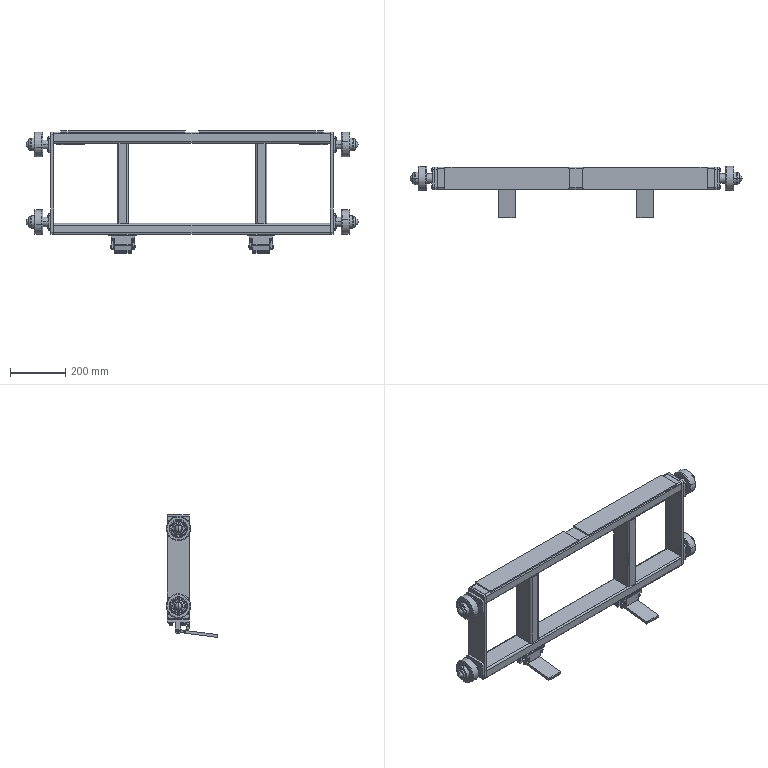Assembly | SolidWorks | mm | 114 component files | 114 solids | 2486 faces | box 1200 x 186.22 x 443.19 mm | volume 4209705 mm3 | cylinder 894 | plane 856 | torus 336 | sphere 224 | cone 176 | commonest cylinder face diameters 10 x84 8 x80 6 x80 4 x52 6.5 x48 9.684 x48 16 x40 11 x32
Bill of materials:
GB_T70.1-2000_SocketHeadCapScrew_M6_16 | 16 |  | Headed pin or screw-like body: a short, larger-diameter cylindrical head joined to a longer, smaller-diameter plain cylindrical shank that has a chamfered free end.
GB_T70.1-2000_SocketHeadCapScrew_M8_25 | 8 |  | Headed cylindrical body: a short, wide cylindrical head with a longer, narrower plain cylindrical shank that has a chamfered end. The shape is very close to the previous part, with slightly different proportions.
GB_T93-1987StandardTypeSpringWasher(Assembly)6x1.6 | 16 |  | Split ring with a rectangular cross-section and a single radial gap. Its radial width is fairly large compared with its thickness, which suggests a split-washer shape.
GB_T93-1987StandardTypeSpringWasher(Assembly)8x2.1 | 8 |  | Flat split ring: a thin annulus with one narrow radial slot cut through it, and a rectangular cross-section.
GB_T97.2-1985FlatWasherChamferedTypeA8x1.6 | 8 | Steel | Flat washer-like annulus: a thin disc with a central circular hole, chamfered on one outer edge.
GB_T276-94DeepGrooveBallBearing6305-2Z | 4 |  | Ring assembly-like solid that looks like a radial ball bearing: concentric outer and inner rings with a central bore, and several spherical elements visible in the annular gap between them.
GB893.2-86RetainingRingForHolesTypeB62 | 4 |  | Thin open ring shaped like an internal retaining ring: a circular band with an opening at one side, ending in two widened lugs that each have a small hole.
GuideWheel | 4 | Nylon 101 | Plain thick ring or sleeve: a wide annulus with a large central bore and rounded outer edges.
GuideWheelAxis | 4 | Q235 | Stepped solid cylinder or shaft: a larger-diameter central section with smaller-diameter end sections on both sides, one longer than the other, both with chamfered ends.
GuideWheelBracketPlate | 4 | Q235 | Flat rectangular plate with rounded corners, a large central circular through hole, and four smaller through holes near the corners.
WD-03UniversalBall | 4 |  | Compound axisymmetric body: a domed or hemispherical end, a stepped cylindrical housing with a wider collar band, and a small cylindrical pin with a chamfered tip projecting from the opposite face.
AWS5_30 | 4 |  | Long, thin-walled hollow cylindrical body with an open, nearly circular round-wire hook loop at each end. The hooks sit on the body axis and look like they lie in the same plane. Overall it looks like a simplified extension spring with the coils drawn as a smooth tube.
GB_T70.1-2000_SocketHeadCapScrew_M4_12 | 8 |  | Socket-head-style headed body: a cylindrical head with a hexagonal recess in its end face, and a plain cylindrical shank with a chamfered tip.
GB_T78-2000HexagonSocketConePointSetScrewM4x6 | 4 |  | Short solid cylinder with a conical top that ends in a small flat circular tip and a chamfer around the bottom edge.
LiftingPlate | 2 | Plain Carbon Steel | Flat rectangular leaf with a hollow cylindrical knuckle (bored boss) along one edge and a small hole near the knuckle. The free end is slightly rounded.
LiftingPlateAxis | 2 | Plain Carbon Steel | Straight solid cylindrical rod or pin with small chamfers at both ends.
LiftingPlateBracket | 2 | Plain Carbon Steel | Bracket block: a rectangular top plate with four corner through holes and downward legs or lugs below it. One lug has a large cross bore and chamfered lower corners. A narrower leg has a small conical-bottom hole.
RectangularTubeEndPlate | 2 | Plain Carbon Steel | Thin, elongated rectangular plate with rounded corners and eight small holes arranged in two groups of four, one group near each end.
RectangularTubeWeldPlate1 | 2 | Plain Carbon Steel | Flat rectangular plate, close to square, with rounded corners and four through holes near the corners.
RectangularTubeWeldPlate2 | 2 | Plain Carbon Steel | Thin, long rectangular strip or plate with small rounded corners and no holes.
RectangularTubeWeldPlate3 | 2 | Plain Carbon Steel | Flat rectangular plate with rounded corners and four through holes near the corners. It is more elongated than unnamed part.
VerticalMovingRectangularTube | 2 | Plain Carbon Steel | Long, straight, hollow rectangular tube with rounded corners and a thin uniform wall. The ends are cut square.
VerticalMovingTube | 2 | Plain Carbon Steel | Short, hollow rectangular tube with rounded corners and a thin uniform wall. The cross-section is about 1:2 and the ends are open and cut square.
Mates:
1. coincident | VerticalMovingRectangularTubeWeldment-1/RectangularTubeWeldPlate1-1 face at (510, 56.339, -25) dir (0, 0, -1) | LiftingPlateAssembly-1/LiftingPlateBracket-1 face at (-207.5, -40, -25) dir (0, 0, 1)
2. concentric | VerticalMovingRectangularTubeWeldment-1/RectangularTubeWeldPlate1-1 face at (-280, 27.5, -25) dir (0, 0, -1) r 4 | LiftingPlateAssembly-1/LiftingPlateBracket-1 face at (-280, 27.5, -35) dir (0, 0, -1) r 4.5
3. concentric | VerticalMovingRectangularTubeWeldment-1/RectangularTubeWeldPlate1-1 face at (-220, -19, -25) dir (0, 0, -1) r 4 | LiftingPlateAssembly-1/LiftingPlateBracket-1 face at (-220, -19, -35) dir (0, 0, -1) r 4.5
4. coincident | VerticalMovingRectangularTubeWeldment-1/RectangularTubeWeldPlate1-2 face at (510, 56.339, -25) dir (0, 0, -1) | LiftingPlateAssembly-2/LiftingPlateBracket-1 face at (292.5, -40, -25) dir (0, 0, 1)
5. concentric | VerticalMovingRectangularTubeWeldment-1/RectangularTubeWeldPlate1-2 face at (220, 27.5, -25) dir (0, 0, -1) r 4 | LiftingPlateAssembly-2/LiftingPlateBracket-1 face at (220, 27.5, -35) dir (0, 0, -1) r 4.5
6. concentric | VerticalMovingRectangularTubeWeldment-1/RectangularTubeWeldPlate1-2 face at (280, -19, -25) dir (0, 0, -1) r 4 | LiftingPlateAssembly-2/LiftingPlateBracket-1 face at (280, -19, -35) dir (0, 0, -1) r 4.5
7. coincident | VerticalMovingRectangularTubeWeldment-1/RectangularTubeEndPlate-1 face at (-510, 0, 165) dir (-1, 0, 0) | GuideWheelAssembly-1/GuideWheelBracket-1/GuideWheelBracketPlate-1 face at (-510, 0, 25) dir (1, 0, 0)
8. concentric | VerticalMovingRectangularTubeWeldment-1/RectangularTubeEndPlate-1 face at (-510, 30, 5) dir (-1, 0, 0) r 3 | GuideWheelAssembly-1/GuideWheelBracket-1/GuideWheelBracketPlate-1 face at (-520, 30, 5) dir (-1, 0, 0) r 5.5
9. concentric | VerticalMovingRectangularTubeWeldment-1/RectangularTubeEndPlate-1 face at (-510, -30, 45) dir (-1, 0, 0) r 3 | GuideWheelAssembly-1/GuideWheelBracket-1/GuideWheelBracketPlate-1 face at (-520, -30, 45) dir (-1, 0, 0) r 5.5
10. coincident | VerticalMovingRectangularTubeWeldment-1/RectangularTubeEndPlate-1 face at (-510, 0, 165) dir (-1, 0, 0) | GuideWheelAssembly-2/GuideWheelBracket-1/GuideWheelBracketPlate-1 face at (-510, 0, 305) dir (1, 0, 0)
11. concentric | VerticalMovingRectangularTubeWeldment-1/RectangularTubeEndPlate-1 face at (-510, 30, 325) dir (-1, 0, 0) r 3 | GuideWheelAssembly-2/GuideWheelBracket-1/GuideWheelBracketPlate-1 face at (-520, 30, 325) dir (-1, 0, 0) r 5.5
12. concentric | VerticalMovingRectangularTubeWeldment-1/RectangularTubeEndPlate-1 face at (-510, -30, 285) dir (-1, 0, 0) r 3 | GuideWheelAssembly-2/GuideWheelBracket-1/GuideWheelBracketPlate-1 face at (-520, -30, 285) dir (-1, 0, 0) r 5.5
13. coincident | VerticalMovingRectangularTubeWeldment-1/RectangularTubeEndPlate-2 face at (510, 0, 165) dir (1, 0, 0) | GuideWheelAssembly-3/GuideWheelBracket-1/GuideWheelBracketPlate-1 face at (510, 0, 25) dir (-1, 0, 0)
14. concentric | VerticalMovingRectangularTubeWeldment-1/RectangularTubeEndPlate-2 face at (510, 30, 45) dir (1, 0, 0) r 3 | GuideWheelAssembly-3/GuideWheelBracket-1/GuideWheelBracketPlate-1 face at (520, 30, 45) dir (1, 0, 0) r 5.5
15. concentric | VerticalMovingRectangularTubeWeldment-1/RectangularTubeEndPlate-2 face at (510, -30, 5) dir (1, 0, 0) r 3 | GuideWheelAssembly-3/GuideWheelBracket-1/GuideWheelBracketPlate-1 face at (520, -30, 5) dir (1, 0, 0) r 5.5
16. coincident | VerticalMovingRectangularTubeWeldment-1/RectangularTubeEndPlate-2 face at (510, 0, 165) dir (1, 0, 0) | GuideWheelAssembly-4/GuideWheelBracket-1/GuideWheelBracketPlate-1 face at (510, 0, 305) dir (-1, 0, 0)
17. concentric | VerticalMovingRectangularTubeWeldment-1/RectangularTubeEndPlate-2 face at (510, 30, 325) dir (1, 0, 0) r 3 | GuideWheelAssembly-4/GuideWheelBracket-1/GuideWheelBracketPlate-1 face at (520, 30, 325) dir (1, 0, 0) r 5.5
18. concentric | VerticalMovingRectangularTubeWeldment-1/RectangularTubeEndPlate-2 face at (510, -30, 285) dir (1, 0, 0) r 3 | GuideWheelAssembly-4/GuideWheelBracket-1/GuideWheelBracketPlate-1 face at (520, -30, 285) dir (1, 0, 0) r 5.5
19. coincident | GuideWheelAssembly-2/GuideWheelBracket-1/GuideWheelBracketPlate-1 face at (-513.2, 26.7, 325) dir (-1, 0, 0) | GB_T93-1987StandardTypeSpringWasher(Assembly)6x1.6-1 face at (-513.2, 30, 325) dir (1, 0, 0)
20. coincident | GuideWheelAssembly-2/GuideWheelBracket-1/GuideWheelBracketPlate-1 face at (-513.2, 26.7, 325) dir (-1, 0, 0) | GB_T93-1987StandardTypeSpringWasher(Assembly)6x1.6-15 face at (-513.2, -30, 325) dir (1, 0, 0)
21. concentric | GuideWheelAssembly-2/GuideWheelBracket-1/GuideWheelBracketPlate-1 face at (-520, 30, 325) dir (-1, 0, 0) r 5.5 | GB_T93-1987StandardTypeSpringWasher(Assembly)6x1.6-1 face at (-513.2, 30, 325) dir (-1, 0, 0) r 3.25
22. concentric | GuideWheelAssembly-2/GuideWheelBracket-1/GuideWheelBracketPlate-1 face at (-520, -30, 325) dir (-1, 0, 0) r 5.5 | GB_T93-1987StandardTypeSpringWasher(Assembly)6x1.6-15 face at (-513.2, -30, 325) dir (-1, 0, 0) r 3.25
23. coincident | GuideWheelAssembly-4/GuideWheelBracket-1/GuideWheelBracketPlate-1 face at (513.2, 33.3, 325) dir (1, 0, 0) | GB_T93-1987StandardTypeSpringWasher(Assembly)6x1.6-19 face at (513.2, 30, 325) dir (-1, 0, 0)
24. coincident | GuideWheelAssembly-4/GuideWheelBracket-1/GuideWheelBracketPlate-1 face at (513.2, 33.3, 325) dir (1, 0, 0) | GB_T93-1987StandardTypeSpringWasher(Assembly)6x1.6-23 face at (513.2, -30, 325) dir (-1, 0, 0)
25. concentric | GuideWheelAssembly-4/GuideWheelBracket-1/GuideWheelBracketPlate-1 face at (520, 30, 325) dir (1, 0, 0) r 5.5 | GB_T93-1987StandardTypeSpringWasher(Assembly)6x1.6-19 face at (513.2, 30, 325) dir (1, 0, 0) r 3.25
26. concentric | GuideWheelAssembly-4/GuideWheelBracket-1/GuideWheelBracketPlate-1 face at (520, -30, 325) dir (1, 0, 0) r 5.5 | GB_T93-1987StandardTypeSpringWasher(Assembly)6x1.6-23 face at (513.2, -30, 325) dir (1, 0, 0) r 3.25
27. coincident | GB_T93-1987StandardTypeSpringWasher(Assembly)6x1.6-1 face at (-514.8, 30, 325) dir (-1, 0, 0) | GB_T70.1-2000_SocketHeadCapScrew_M6_16-15 face at (-514.8, 35, 325) dir (1, 0, 0)
28. coincident | GB_T70.1-2000_SocketHeadCapScrew_M6_16-1 face at (-514.8, -25, 325) dir (1, 0, 0) | GB_T70.1-2000_SocketHeadCapScrew_M6_16-15 face at (-514.8, 35, 325) dir (1, 0, 0)
29. concentric | GuideWheelAssembly-2/GuideWheelBracket-1/GuideWheelBracketPlate-1 face at (-520, 30, 325) dir (-1, 0, 0) r 5.5 | GB_T70.1-2000_SocketHeadCapScrew_M6_16-15 face at (-520.8, 30, 325) dir (-1, 0, 0) r 3
30. concentric | GuideWheelAssembly-2/GuideWheelBracket-1/GuideWheelBracketPlate-1 face at (-520, -30, 325) dir (-1, 0, 0) r 5.5 | GB_T70.1-2000_SocketHeadCapScrew_M6_16-1 face at (-520.8, -30, 325) dir (-1, 0, 0) r 3
31. coincident | GB_T93-1987StandardTypeSpringWasher(Assembly)6x1.6-23 face at (514.8, -30, 325) dir (1, 0, 0) | GB_T70.1-2000_SocketHeadCapScrew_M6_16-19 face at (514.8, 31.909, 320.379) dir (-1, 0, 0)
32. coincident | GB_T93-1987StandardTypeSpringWasher(Assembly)6x1.6-23 face at (514.8, -30, 325) dir (1, 0, 0) | GB_T70.1-2000_SocketHeadCapScrew_M6_16-23 face at (514.8, -28.091, 320.379) dir (-1, 0, 0)
33. concentric | GuideWheelAssembly-4/GuideWheelBracket-1/GuideWheelBracketPlate-1 face at (520, -30, 325) dir (1, 0, 0) r 5.5 | GB_T70.1-2000_SocketHeadCapScrew_M6_16-23 face at (520.8, -30, 325) dir (1, 0, 0) r 3
34. concentric | GuideWheelAssembly-4/GuideWheelBracket-1/GuideWheelBracketPlate-1 face at (520, 30, 325) dir (1, 0, 0) r 5.5 | GB_T70.1-2000_SocketHeadCapScrew_M6_16-19 face at (520.8, 30, 325) dir (1, 0, 0) r 3
35. coincident | LiftingPlateAssembly-1/LiftingPlateBracket-1 face at (-207.5, 12, -35) dir (0, 0, -1) | GB_T97.2-1985FlatWasherChamferedTypeA8x1.6-13 face at (-284.2, -19, -35) dir (0, 0, 1)
36. coincident | LiftingPlateAssembly-1/LiftingPlateBracket-1 face at (-207.5, -8, -35) dir (0, 0, -1) | GB_T97.2-1985FlatWasherChamferedTypeA8x1.6-11 face at (-224.2, 27.5, -35) dir (0, 0, 1)
37. coincident | LiftingPlateAssembly-1/LiftingPlateBracket-1 face at (-207.5, -8, -35) dir (0, 0, -1) | GB_T97.2-1985FlatWasherChamferedTypeA8x1.6-9 face at (-224.2, -19, -35) dir (0, 0, 1)
38. coincident | LiftingPlateAssembly-1/LiftingPlateBracket-1 face at (-207.5, -8, -35) dir (0, 0, -1) | GB_T97.2-1985FlatWasherChamferedTypeA8x1.6-1 face at (-284.2, 27.5, -35) dir (0, 0, 1)
39. concentric | LiftingPlateAssembly-1/LiftingPlateBracket-1 face at (-280, -19, -35) dir (0, 0, -1) r 4.5 | GB_T97.2-1985FlatWasherChamferedTypeA8x1.6-13 face at (-280, -19, -26.355) dir (0, 0, 1) r 4.2
40. concentric | LiftingPlateAssembly-1/LiftingPlateBracket-1 face at (-280, 27.5, -35) dir (0, 0, -1) r 4.5 | GB_T97.2-1985FlatWasherChamferedTypeA8x1.6-1 face at (-280, 27.5, -26.355) dir (0, 0, 1) r 4.2
41. concentric | LiftingPlateAssembly-1/LiftingPlateBracket-1 face at (-220, 27.5, -35) dir (0, 0, -1) r 4.5 | GB_T97.2-1985FlatWasherChamferedTypeA8x1.6-11 face at (-220, 27.5, -26.355) dir (0, 0, 1) r 4.2
42. concentric | LiftingPlateAssembly-1/LiftingPlateBracket-1 edge at (-220, -19, -35) dir (0, 0, -1) r 4.5 | GB_T97.2-1985FlatWasherChamferedTypeA8x1.6-9 face at (-220, -19, -26.355) dir (0, 0, 1) r 4.2
43. coincident | GB_T97.2-1985FlatWasherChamferedTypeA8x1.6-13 face at (-284.2, -19, -36.6) dir (0, 0, -1) | GB_T93-1987StandardTypeSpringWasher(Assembly)8x2.1-8 face at (-280, -19, -36.6) dir (0, 0, 1)
44. coincident | GB_T93-1987StandardTypeSpringWasher(Assembly)8x2.1-6 face at (-220, 27.5, -36.6) dir (0, 0, 1) | GB_T93-1987StandardTypeSpringWasher(Assembly)8x2.1-8 face at (-280, -19, -36.6) dir (0, 0, 1)
45. coincident | GB_T93-1987StandardTypeSpringWasher(Assembly)8x2.1-8 face at (-280, -19, -36.6) dir (0, 0, 1) | GB_T93-1987StandardTypeSpringWasher(Assembly)8x2.1-10 face at (-280, 27.5, -36.6) dir (0, 0, 1)
46. coincident | GB_T93-1987StandardTypeSpringWasher(Assembly)8x2.1-1 face at (-220, -19, -36.6) dir (0, 0, 1) | GB_T93-1987StandardTypeSpringWasher(Assembly)8x2.1-6 face at (-220, 27.5, -36.6) dir (0, 0, 1)
47. concentric | GB_T97.2-1985FlatWasherChamferedTypeA8x1.6-11 face at (-220, 27.5, -26.355) dir (0, 0, 1) r 4.2 | GB_T93-1987StandardTypeSpringWasher(Assembly)8x2.1-6 face at (-220, 27.5, -36.6) dir (0, 0, -1) r 4.25
48. concentric | GB_T97.2-1985FlatWasherChamferedTypeA8x1.6-1 face at (-280, 27.5, -26.355) dir (0, 0, 1) r 4.2 | GB_T93-1987StandardTypeSpringWasher(Assembly)8x2.1-10 face at (-280, 27.5, -36.6) dir (0, 0, -1) r 4.25
49. concentric | GB_T97.2-1985FlatWasherChamferedTypeA8x1.6-13 face at (-280, -19, -26.355) dir (0, 0, 1) r 4.2 | GB_T93-1987StandardTypeSpringWasher(Assembly)8x2.1-8 face at (-280, -19, -36.6) dir (0, 0, -1) r 4.25
50. concentric | GB_T97.2-1985FlatWasherChamferedTypeA8x1.6-9 face at (-220, -19, -26.355) dir (0, 0, 1) r 4.2 | GB_T93-1987StandardTypeSpringWasher(Assembly)8x2.1-1 face at (-220, -19, -36.6) dir (0, 0, -1) r 4.25
51. coincident | GB_T93-1987StandardTypeSpringWasher(Assembly)8x2.1-10 face at (-280, 27.5, -38.2) dir (0, 0, -1) | GB_T70.1-2000_SocketHeadCapScrew_M8_25-8 face at (-280, -12.5, -38.2) dir (0, 0, 1)
52. coincident | GB_T93-1987StandardTypeSpringWasher(Assembly)8x2.1-1 face at (-220, -19, -38.2) dir (0, 0, -1) | GB_T70.1-2000_SocketHeadCapScrew_M8_25-12 face at (-220, -12.5, -38.2) dir (0, 0, 1)
53. coincident | GB_T93-1987StandardTypeSpringWasher(Assembly)8x2.1-1 face at (-220, -19, -38.2) dir (0, 0, -1) | GB_T70.1-2000_SocketHeadCapScrew_M8_25-1 face at (-220, 34, -38.2) dir (0, 0, 1)
54. coincident | GB_T93-1987StandardTypeSpringWasher(Assembly)8x2.1-1 face at (-220, -19, -38.2) dir (0, 0, -1) | GB_T70.1-2000_SocketHeadCapScrew_M8_25-10 face at (-280, 34, -38.2) dir (0, 0, 1)
55. concentric | GB_T93-1987StandardTypeSpringWasher(Assembly)8x2.1-1 face at (-220, -19, -36.6) dir (0, 0, -1) r 4.25 | GB_T70.1-2000_SocketHeadCapScrew_M8_25-12 face at (-220, -19, -46.2) dir (0, 0, -1) r 4
56. concentric | GB_T93-1987StandardTypeSpringWasher(Assembly)8x2.1-6 face at (-220, 27.5, -36.6) dir (0, 0, -1) r 4.25 | GB_T70.1-2000_SocketHeadCapScrew_M8_25-1 face at (-220, 27.5, -46.2) dir (0, 0, -1) r 4
57. concentric | GB_T93-1987StandardTypeSpringWasher(Assembly)8x2.1-10 face at (-280, 27.5, -36.6) dir (0, 0, -1) r 4.25 | GB_T70.1-2000_SocketHeadCapScrew_M8_25-10 face at (-280, 27.5, -46.2) dir (0, 0, -1) r 4
58. concentric | GB_T93-1987StandardTypeSpringWasher(Assembly)8x2.1-8 face at (-280, -19, -36.6) dir (0, 0, -1) r 4.25 | GB_T70.1-2000_SocketHeadCapScrew_M8_25-8 face at (-280, -19, -46.2) dir (0, 0, -1) r 4
59. concentric | GuideWheelBracket-1/GuideWheelAxis-1 face at (0, 0, 54) dir (0, 0, -1) r 12.5 | GB_T276-94DeepGrooveBallBearing6305-2Z-1 face at (0, 0, 57.921) dir (0, 0, 1) r 12.5
60. coincident | GuideWheelBracket-1/GuideWheelAxis-1 face at (0, 0, 37) dir (0, 0, 1) | GB_T276-94DeepGrooveBallBearing6305-2Z-1 face at (0, 18, 37) dir (0, 0, -1)
61. coincident | GuideWheelBracket-1/GuideWheelAxis-1 face at (0, 0, 54) dir (0, 0, 1) | WD-03UniversalBall-1 face at (0, 0, 54) dir (0, 0, -1)
62. concentric | GuideWheelBracket-1/GuideWheelAxis-1 face at (0, 0, 54) dir (0, 0, 1) r 5 | WD-03UniversalBall-1 face at (0, 0, 39) dir (0, 0, 1) r 5
63. coincident | GB_T276-94DeepGrooveBallBearing6305-2Z-1 face at (0, 29.9, 37) dir (0, 0, -1) | GuideWheel-2 face at (0, 0, 37) dir (0, 0, 1)
64. concentric | GB_T276-94DeepGrooveBallBearing6305-2Z-1 face at (0, 0, 45.5) dir (0, 0, 1) r 31 | GuideWheel-2 face at (0, 0, 60) dir (0, 0, -1) r 44
65. coincident | GB893.2-86RetainingRingForHolesTypeB62-1 face at (0, 0, 54) dir (0, 0, -1) | GuideWheel-2 face at (0, 0, 54) dir (0, 0, 1)
66. concentric | GB893.2-86RetainingRingForHolesTypeB62-1 face at (0, 0, 56) dir (0, 0, -1) r 33.1 | GuideWheel-2 face at (0, 0, 60) dir (0, 0, -1) r 44
67. concentric | GuideWheelBracketPlate-1 face at (0, 0, 0) dir (0, 0, 1) r 15 | GuideWheelAxis-1 face at (0, 0, 54) dir (0, 0, -1) r 12.5
68. coincident | GuideWheelBracketPlate-1 face at (0, 0, 10) dir (0, 0, 1) | GuideWheelAxis-1 face at (0, 0, 10) dir (0, 0, -1)
69. concentric | LiftingPlateBracket-1 face at (0, 0, -42.5) dir (0, 0, 1) r 5 | LiftingPlate-1 face at (0, 0, 30) dir (0, 0, -1) r 5.25
70. width | LiftingPlate-1 face at (0, 0, 30) dir (0, 0, 1) | LiftingPlate-1 face at (0, 0, -30) dir (0, 0, -1) | LiftingPlateBracket-1 face at (0, 0, -42.5) dir (0, 0, -1) | LiftingPlateBracket-1 face at (0, 0, 42.5) dir (0, 0, 1)
71. concentric | LiftingPlateBracket-1 face at (0, 0, -42.5) dir (0, 0, 1) r 5 | LiftingPlateAxis-2 face at (0, 0, 44) dir (0, 0, -1) r 5
72. width | LiftingPlateBracket-1 face at (0, 0, 42.5) dir (0, 0, 1) | LiftingPlateBracket-1 face at (0, 0, -42.5) dir (0, 0, -1) | LiftingPlateAxis-2 face at (0, 0, -44) dir (0, 0, -1) | LiftingPlateAxis-2 face at (0, 0, 44) dir (0, 0, 1)
73. concentric | LiftingPlateBracket-1 face at (0, 10, -37.5) dir (0, 1, 0) r 2 | GB_T78-2000HexagonSocketConePointSetScrewM4x6-1 face at (0, 12.41, -37.5) dir (0, 1, 0) r 2
74. tangent | LiftingPlateAxis-2 face at (0, 0, 44) dir (0, 0, -1) r 5 | GB_T78-2000HexagonSocketConePointSetScrewM4x6-1 face at (0, 5, -37.5) dir (0, -1, 0)
75. concentric | LiftingPlateBracket-1 face at (0, 10, 37.5) dir (0, 1, 0) r 2 | GB_T78-2000HexagonSocketConePointSetScrewM4x6-2 face at (0, 12.41, 37.5) dir (0, 1, 0) r 2
76. coincident | GB_T78-2000HexagonSocketConePointSetScrewM4x6-1 face at (1.732, 11, -37.5) dir (0, 1, 0) | GB_T78-2000HexagonSocketConePointSetScrewM4x6-2 face at (1.732, 11, 37.5) dir (0, 1, 0)
77. concentric | LiftingPlateBracket-1 face at (-37, -20, -30) dir (0, 0, -1) r 2 | AWS5_30-1 sketch segment at (-37, -20, -32.5) dir (0, 0, 1) r 2.5
78. concentric | LiftingPlate-1 face at (-24.796, 3.184, -30) dir (0, 0, -1) r 2 | AWS5_30-1 sketch segment at (-24.796, 3.184, -32.5) dir (0, 0, 1) r 2.5
79. concentric | LiftingPlateBracket-1 face at (-37, -20, -30) dir (0, 0, -1) r 2 | GB_T70.1-2000_SocketHeadCapScrew_M4_12-1 face at (-37, -20, -39.5) dir (0, 0, -1) r 2
80. distance | LiftingPlateBracket-1 face at (-32, -4.469, -30) dir (0, 0, -1) | GB_T70.1-2000_SocketHeadCapScrew_M4_12-1 face at (-36.592, -16.524, -35.5) dir (0, 0, 1)
81. tangent | LiftingPlateBracket-1 face at (-32, -4.469, -30) dir (0, 0, -1) | AWS5_30-1 face at (-25.681, 1.503, -32.5) dir (-0.4658, -0.8849, 0) r 2.5
82. concentric | LiftingPlate-1 face at (-24.796, 3.184, -30) dir (0, 0, -1) r 2 | GB_T70.1-2000_SocketHeadCapScrew_M4_12-2 face at (-24.796, 3.184, -39.5) dir (0, 0, -1) r 2
83. distance | LiftingPlate-1 face at (0, 0, -30) dir (0, 0, -1) | GB_T70.1-2000_SocketHeadCapScrew_M4_12-2 face at (-24.796, 6.684, -35.5) dir (0, 0, 1)
84. concentric | LiftingPlate-1 face at (-24.796, 3.184, 30) dir (0, 0, 1) r 2 | AWS5_30-2 sketch segment at (-24.796, 3.184, 32.5) dir (0, 0, 1) r 2.5
85. concentric | LiftingPlateBracket-1 face at (-37, -20, 30) dir (0, 0, 1) r 2 | AWS5_30-2 sketch segment at (-37, -20, 32.5) dir (0, 0, 1) r 2.5
86. tangent | LiftingPlateBracket-1 face at (-32, -3.907, 30) dir (0, 0, 1) | AWS5_30-2 face at (-25.681, 1.503, 32.5) dir (-0.4658, -0.8849, 0) r 2.5
87. concentric | LiftingPlate-1 face at (-24.796, 3.184, 30) dir (0, 0, 1) r 2 | GB_T70.1-2000_SocketHeadCapScrew_M4_12-3 face at (-24.796, 3.184, 39.5) dir (0, 0, 1) r 2
88. distance | LiftingPlate-1 face at (0, 0, 30) dir (0, 0, 1) | GB_T70.1-2000_SocketHeadCapScrew_M4_12-3 face at (-24.796, 6.684, 35.5) dir (0, 0, -1)
89. concentric | LiftingPlateBracket-1 face at (-37, -20, 30) dir (0, 0, 1) r 2 | GB_T70.1-2000_SocketHeadCapScrew_M4_12-4 face at (-37, -20, 39.5) dir (0, 0, 1) r 2
90. distance | LiftingPlateBracket-1 face at (-32, -3.907, 30) dir (0, 0, 1) | GB_T70.1-2000_SocketHeadCapScrew_M4_12-4 face at (-37, -16.5, 35.5) dir (0, 0, -1)
91. coincident | VerticalMovingRectangularTube-1 face at (500, 34, -20) dir (0, 0, -1) | RectangularTubeWeldPlate1-1 face at (-250, 0, -20) dir (0, 0, 1)
92. width | RectangularTubeWeldPlate1-1 face at (-300, 40, -20) dir (0, 1, 0) | RectangularTubeWeldPlate1-1 face at (-300, -40, -20) dir (0, -1, 0) | VerticalMovingRectangularTube-1 face at (500, -40, 14) dir (0, -1, 0) | VerticalMovingRectangularTube-1 face at (500, 40, -14) dir (0, 1, 0)
93. coincident | VerticalMovingRectangularTube-1 face at (500, 34, -20) dir (0, 0, -1) | RectangularTubeWeldPlate1-2 face at (250, 0, -20) dir (0, 0, 1)
94. width | RectangularTubeWeldPlate1-2 face at (200, 40, -20) dir (0, 1, 0) | RectangularTubeWeldPlate1-2 face at (200, -40, -20) dir (0, -1, 0) | VerticalMovingRectangularTube-1 face at (500, -40, 14) dir (0, -1, 0) | VerticalMovingRectangularTube-1 face at (500, 40, -14) dir (0, 1, 0)
95. distance | RectangularTubeWeldPlate1-1 sketch segment at (-250, 40, -20) dir (0, -1, 0) | VerticalMovingRectangularTubeWeldment plane at (0, 0, 0) dir (1, 0, 0)
96. distance | VerticalMovingRectangularTubeWeldment plane at (0, 0, 0) dir (1, 0, 0) | RectangularTubeWeldPlate1-2 sketch segment at (250, 40, -20) dir (0, -1, 0)
97. coincident | VerticalMovingRectangularTube-1 face at (500, -34, 20) dir (0, 0, 1) | VerticalMovingTube-1 face at (-236, 34, 20) dir (0, 0, -1)
98. coincident | VerticalMovingRectangularTube-1 face at (500, 40, -14) dir (0, 1, 0) | VerticalMovingTube-1 face at (-236, 40, 310) dir (0, 1, 0)
99. coincident | VerticalMovingRectangularTube-1 face at (500, -34, 20) dir (0, 0, 1) | VerticalMovingTube-3 face at (264, 34, 20) dir (0, 0, -1)
100. coincident | VerticalMovingRectangularTube-1 face at (500, 40, -14) dir (0, 1, 0) | VerticalMovingTube-3 face at (264, 40, 310) dir (0, 1, 0)
101. coincident | VerticalMovingTube-1 face at (-236, 34, 310) dir (0, 0, 1) | VerticalMovingRectangularTube-4 face at (500, 34, 310) dir (0, 0, -1)
102. coincident | VerticalMovingTube-1 face at (-236, 40, 310) dir (0, 1, 0) | VerticalMovingRectangularTube-4 face at (500, 40, 316) dir (0, 1, 0)
103. coincident | VerticalMovingRectangularTube-1 face at (-500, 34, -14) dir (-1, 0, 0) | VerticalMovingRectangularTube-4 face at (-500, 34, 316) dir (-1, 0, 0)
104. coincident | VerticalMovingRectangularTube-4 face at (500, -34, 350) dir (0, 0, 1) | RectangularTubeWeldPlate2-1 face at (-250, 0, 350) dir (0, 0, -1)
105. coincident | VerticalMovingRectangularTube-4 face at (500, -40, 344) dir (0, -1, 0) | RectangularTubeWeldPlate2-1 face at (-475, -40, 358) dir (0, -1, 0)
106. coincident | VerticalMovingRectangularTube-4 face at (500, -34, 350) dir (0, 0, 1) | RectangularTubeWeldPlate2-2 face at (250, 0, 350) dir (0, 0, -1)
107. coincident | VerticalMovingRectangularTube-4 face at (500, -40, 344) dir (0, -1, 0) | RectangularTubeWeldPlate2-2 face at (25, -40, 358) dir (0, -1, 0)
108. distance | VerticalMovingRectangularTubeWeldment plane at (0, 0, 0) dir (1, 0, 0) | RectangularTubeWeldPlate2-1 sketch segment at (-250, 40, 358) dir (0, -1, 0)
109. distance | VerticalMovingRectangularTubeWeldment plane at (0, 0, 0) dir (1, 0, 0) | RectangularTubeWeldPlate2-2 sketch segment at (250, 40, 358) dir (0, -1, 0)
110. distance | VerticalMovingRectangularTubeWeldment plane at (0, 0, 0) dir (1, 0, 0) | VerticalMovingTube-1 face at (-270, -34, 310) dir (-1, 0, 0)
111. distance | VerticalMovingRectangularTubeWeldment plane at (0, 0, 0) dir (1, 0, 0) | VerticalMovingTube-3 face at (270, 34, 310) dir (1, 0, 0)
112. coincident | VerticalMovingRectangularTube-1 face at (-500, 34, -14) dir (-1, 0, 0) | RectangularTubeEndPlate-1 face at (-500, 0, 165) dir (1, 0, 0)
113. coincident | VerticalMovingRectangularTube-1 face at (500, 34, -20) dir (0, 0, -1) | RectangularTubeEndPlate-1 face at (-510, -40, -20) dir (0, 0, -1)
114. coincident | VerticalMovingRectangularTube-1 face at (500, 40, -14) dir (0, 1, 0) | RectangularTubeEndPlate-1 face at (-510, 40, -20) dir (0, 1, 0)
115. coincident | VerticalMovingRectangularTube-1 face at (500, 34, -14) dir (1, 0, 0) | RectangularTubeEndPlate-2 face at (500, 0, 165) dir (-1, 0, 0)
116. coincident | VerticalMovingRectangularTube-1 face at (500, 40, -14) dir (0, 1, 0) | RectangularTubeEndPlate-2 face at (510, 40, 350) dir (0, 1, 0)
117. coincident | VerticalMovingRectangularTube-1 face at (500, 34, -20) dir (0, 0, -1) | RectangularTubeEndPlate-2 face at (510, -40, -20) dir (0, 0, -1)
118. coincident | VerticalMovingRectangularTube-4 face at (500, 34, 310) dir (0, 0, -1) | RectangularTubeWeldPlate3-1 face at (440, 0, 310) dir (0, 0, 1)
119. distance | RectangularTubeWeldPlate3-1 face at (490, 30, 310) dir (1, 0, 0) | RectangularTubeEndPlate-2 face at (500, 0, 165) dir (-1, 0, 0)
120. width | VerticalMovingRectangularTube-4 face at (500, 40, 316) dir (0, 1, 0) | VerticalMovingRectangularTube-4 face at (500, -40, 344) dir (0, -1, 0) | RectangularTubeWeldPlate3-1 face at (390, -30, 310) dir (0, -1, 0) | RectangularTubeWeldPlate3-1 face at (390, 30, 310) dir (0, 1, 0)
121. coincident | VerticalMovingRectangularTube-4 face at (500, 34, 310) dir (0, 0, -1) | RectangularTubeWeldPlate3-2 face at (-440, 0, 310) dir (0, 0, 1)
122. distance | RectangularTubeEndPlate-1 face at (-500, 0, 165) dir (1, 0, 0) | RectangularTubeWeldPlate3-2 face at (-490, 30, 310) dir (-1, 0, 0)
123. width | RectangularTubeWeldPlate3-2 face at (-490, 30, 310) dir (0, 1, 0) | RectangularTubeWeldPlate3-2 face at (-490, -30, 310) dir (0, -1, 0) | VerticalMovingRectangularTube-4 face at (500, 40, 316) dir (0, 1, 0) | VerticalMovingRectangularTube-4 face at (500, -40, 344) dir (0, -1, 0)